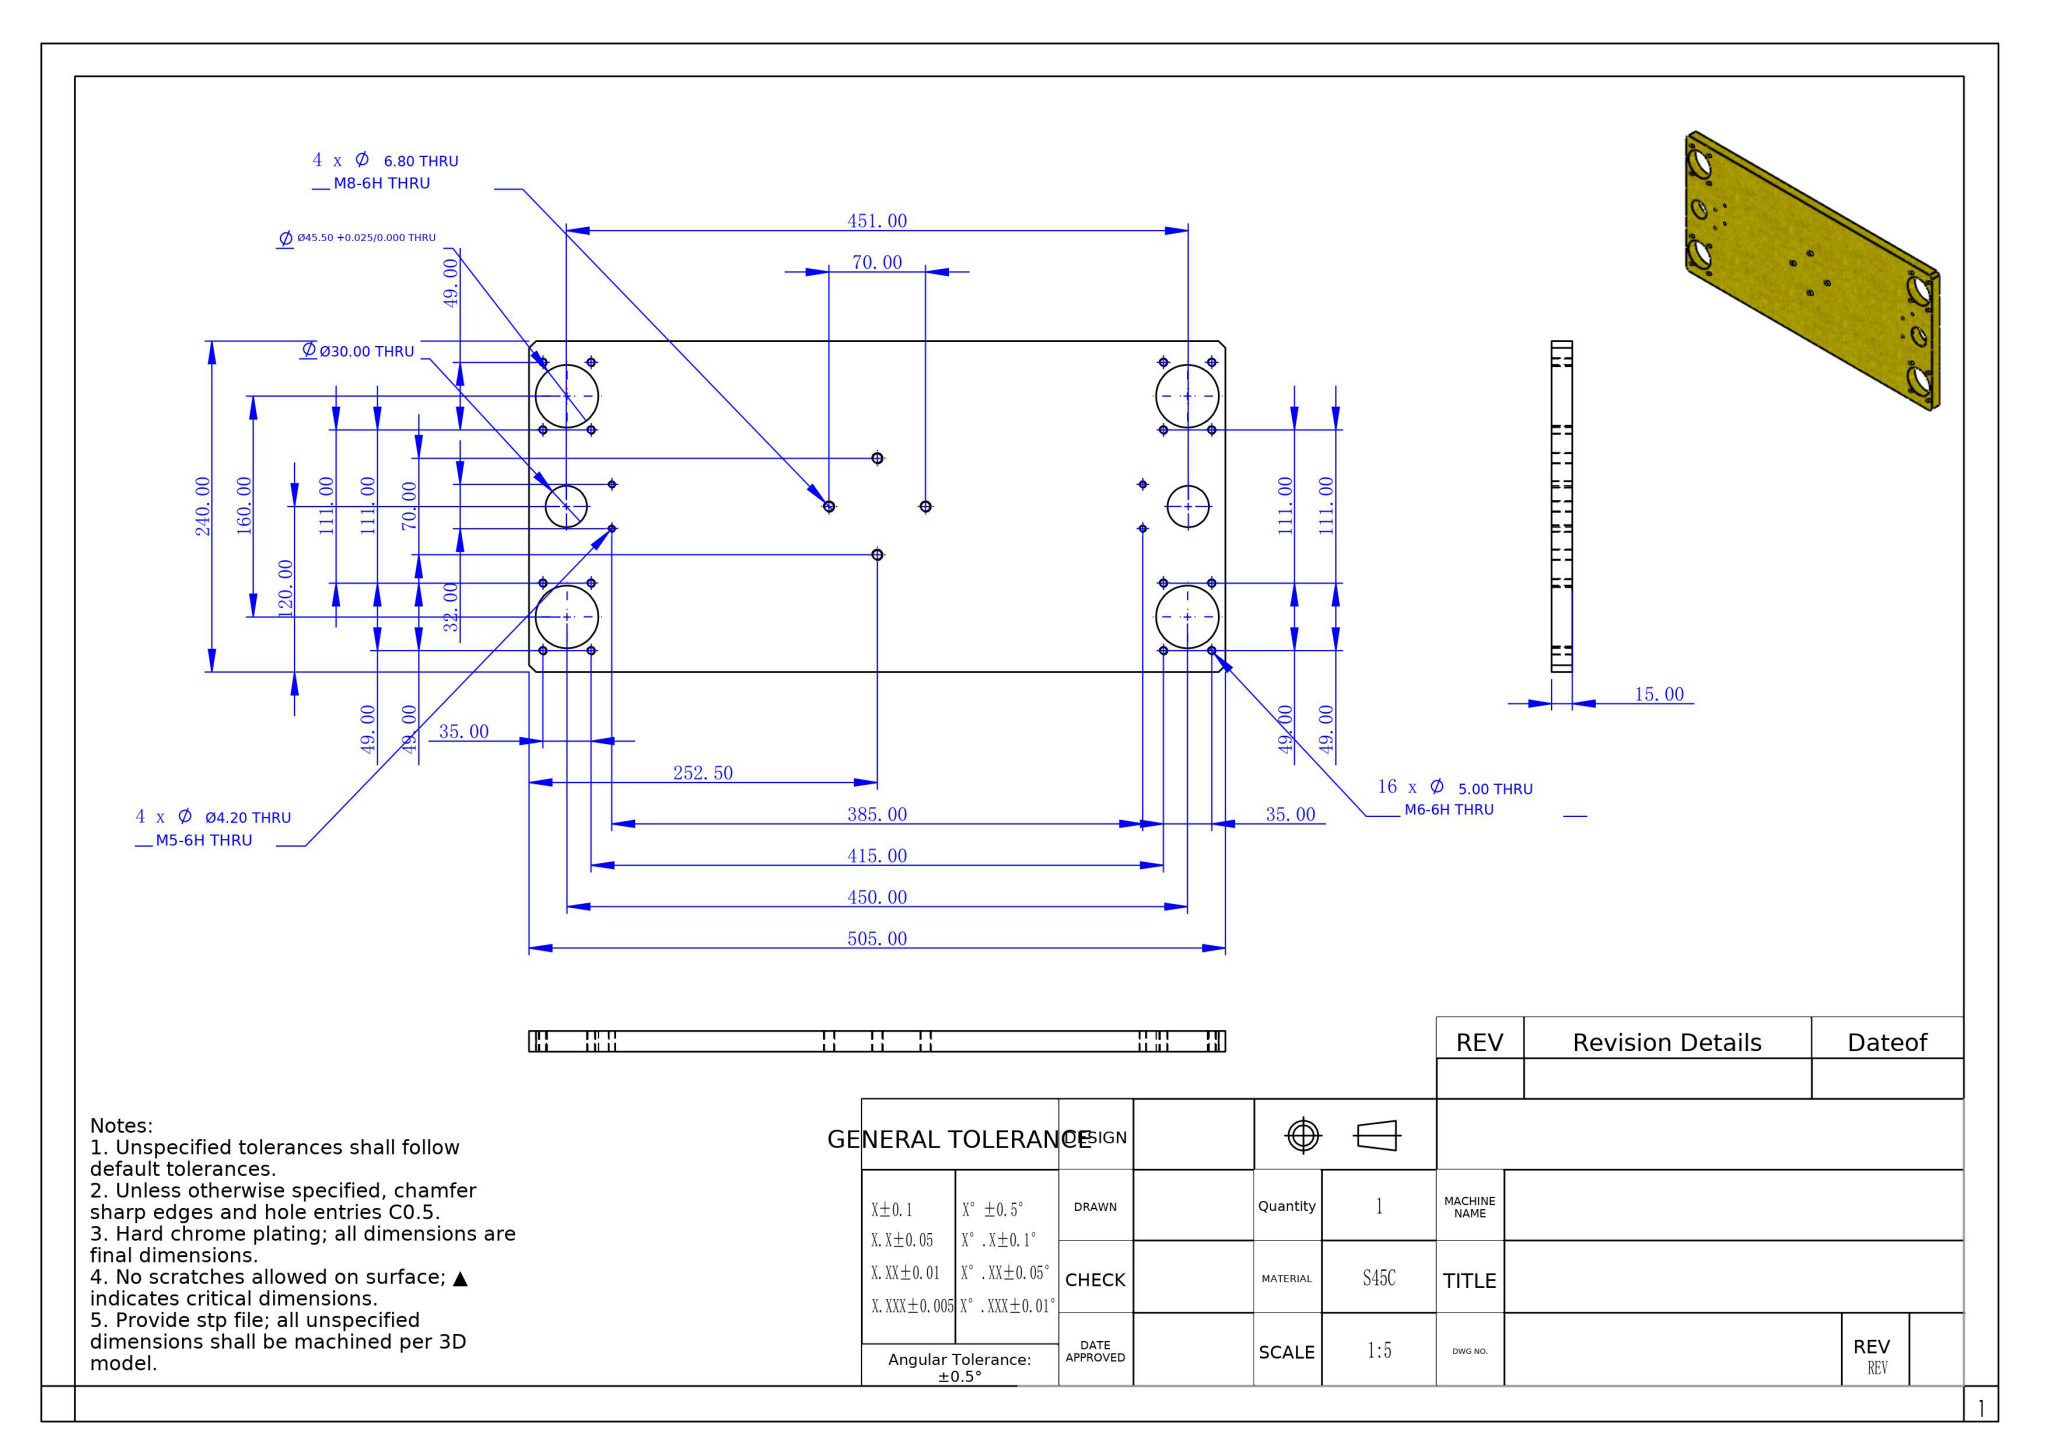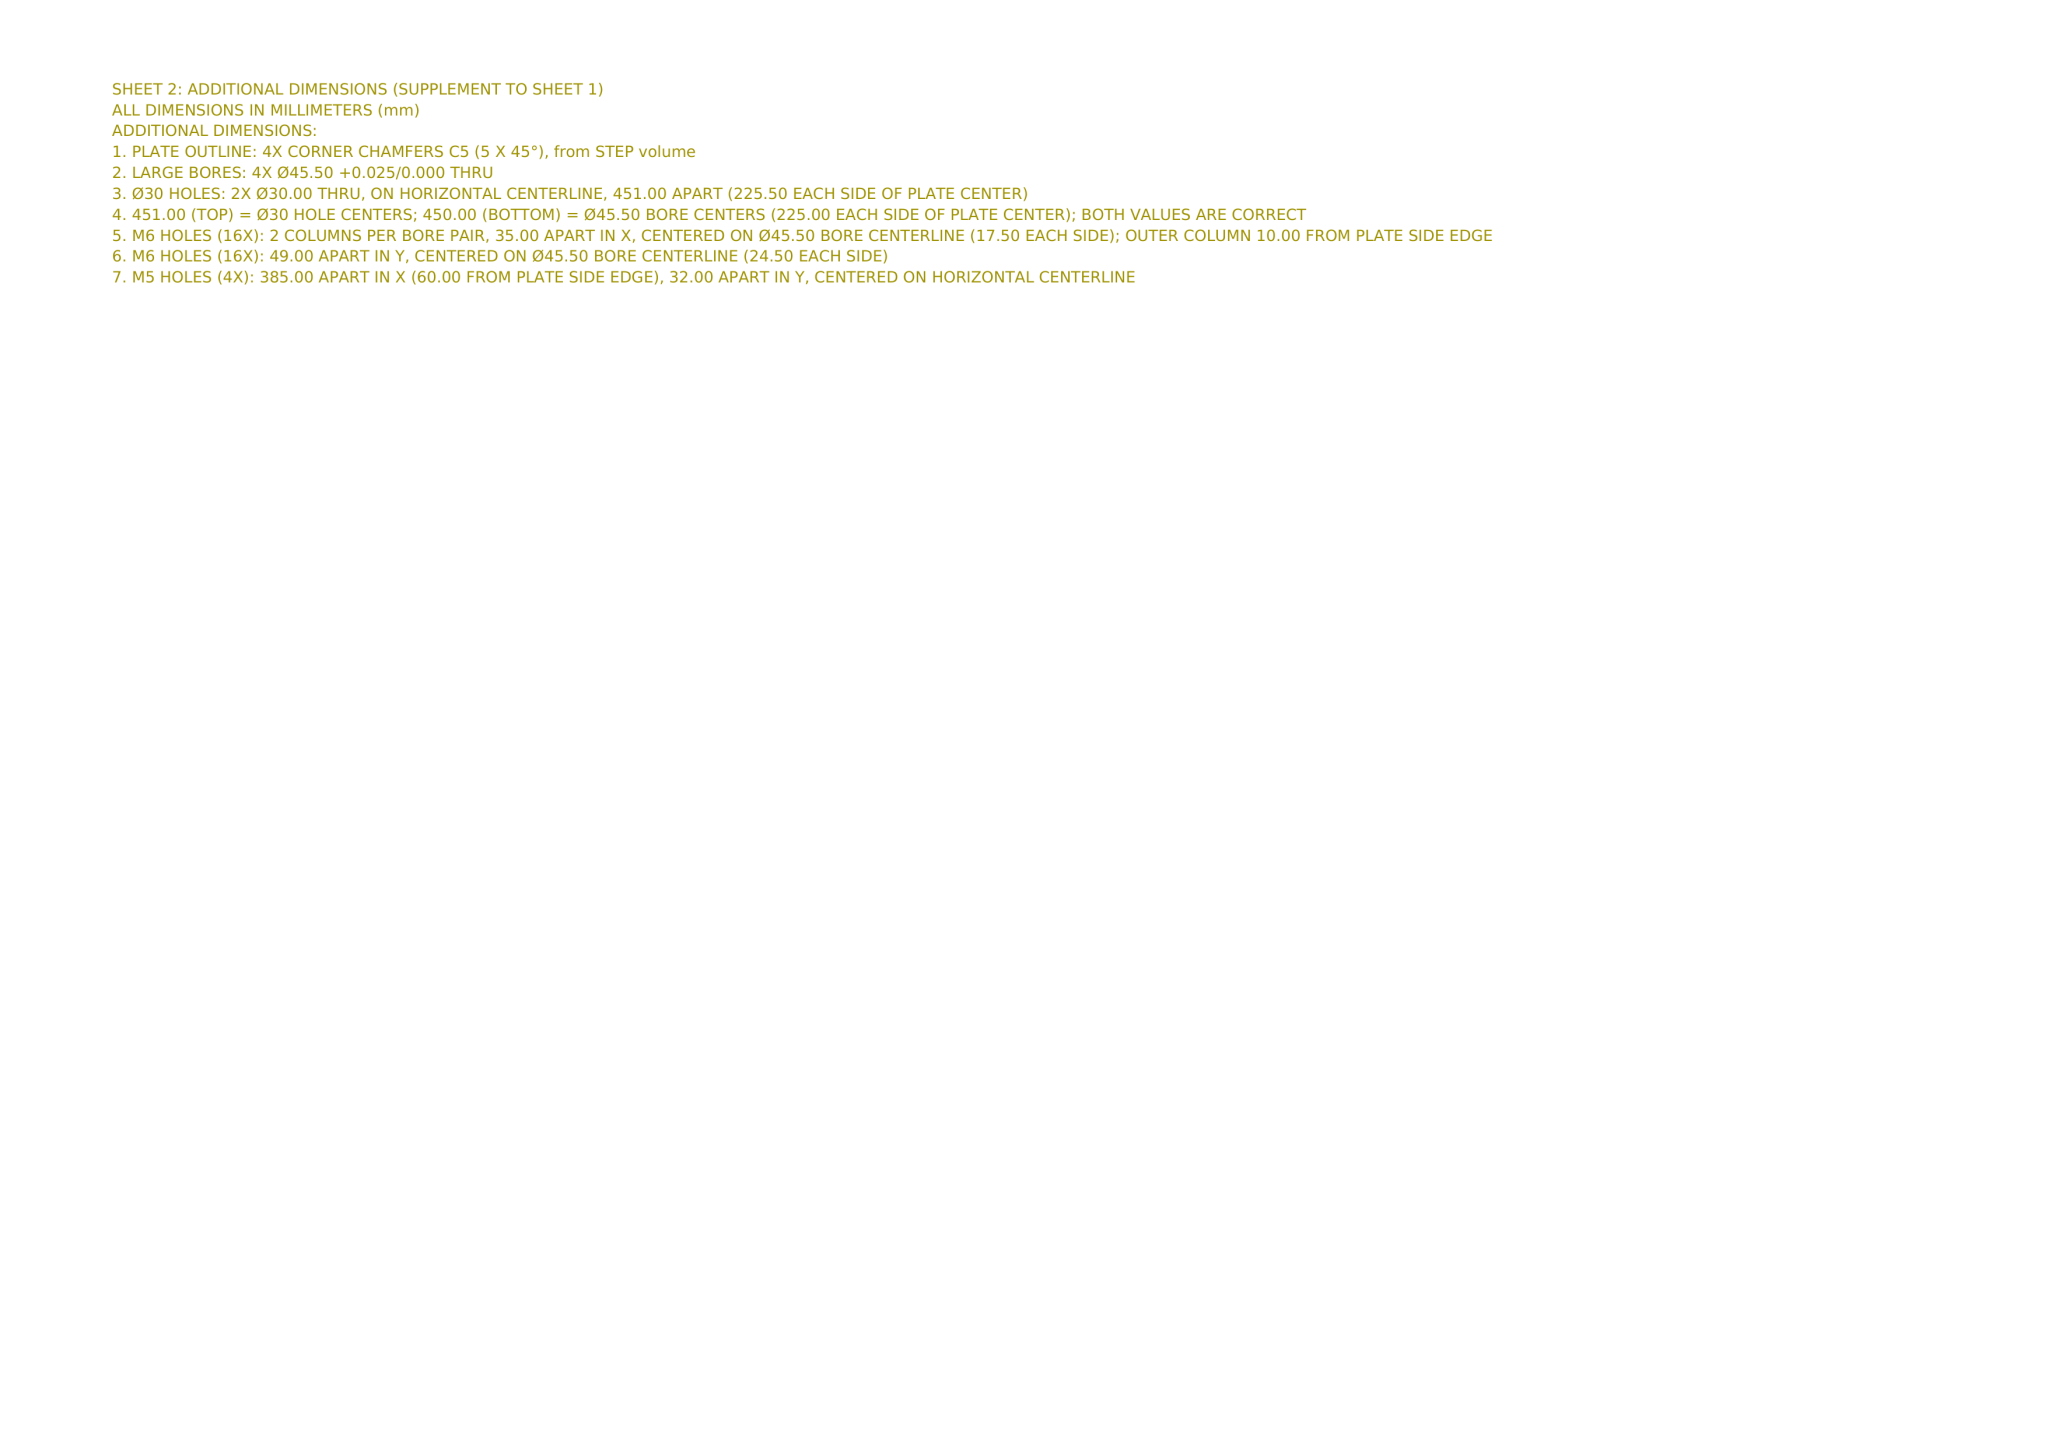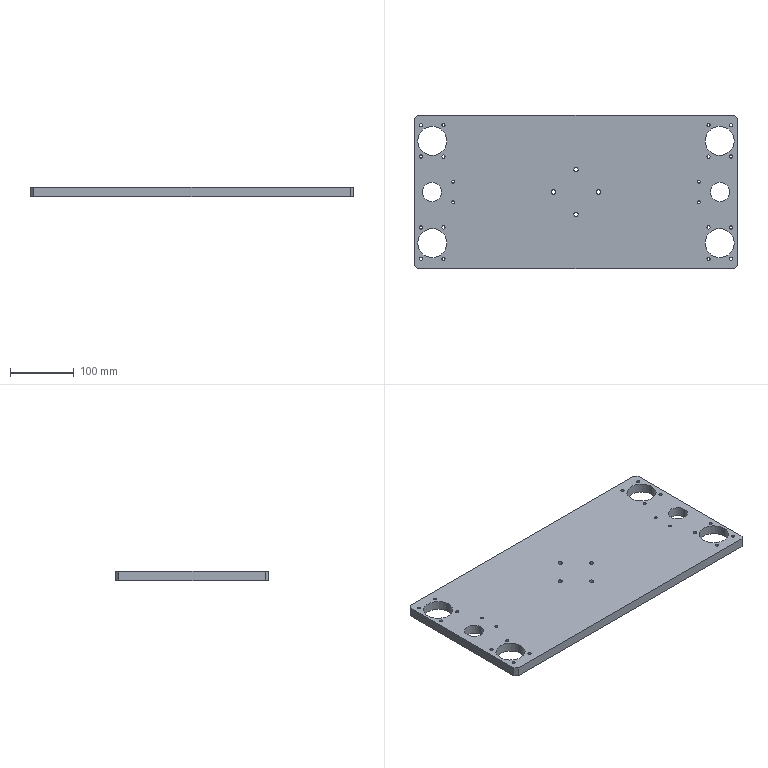Part | NX | mm | 1 solid | 70 faces | box 505 x 240 x 15 mm | volume 1690763 mm3 | cylinder 60 | plane 10 | commonest cylinder face diameters 5 x32 4.2 x8 6.8 x8 45.5 x8 30 x4